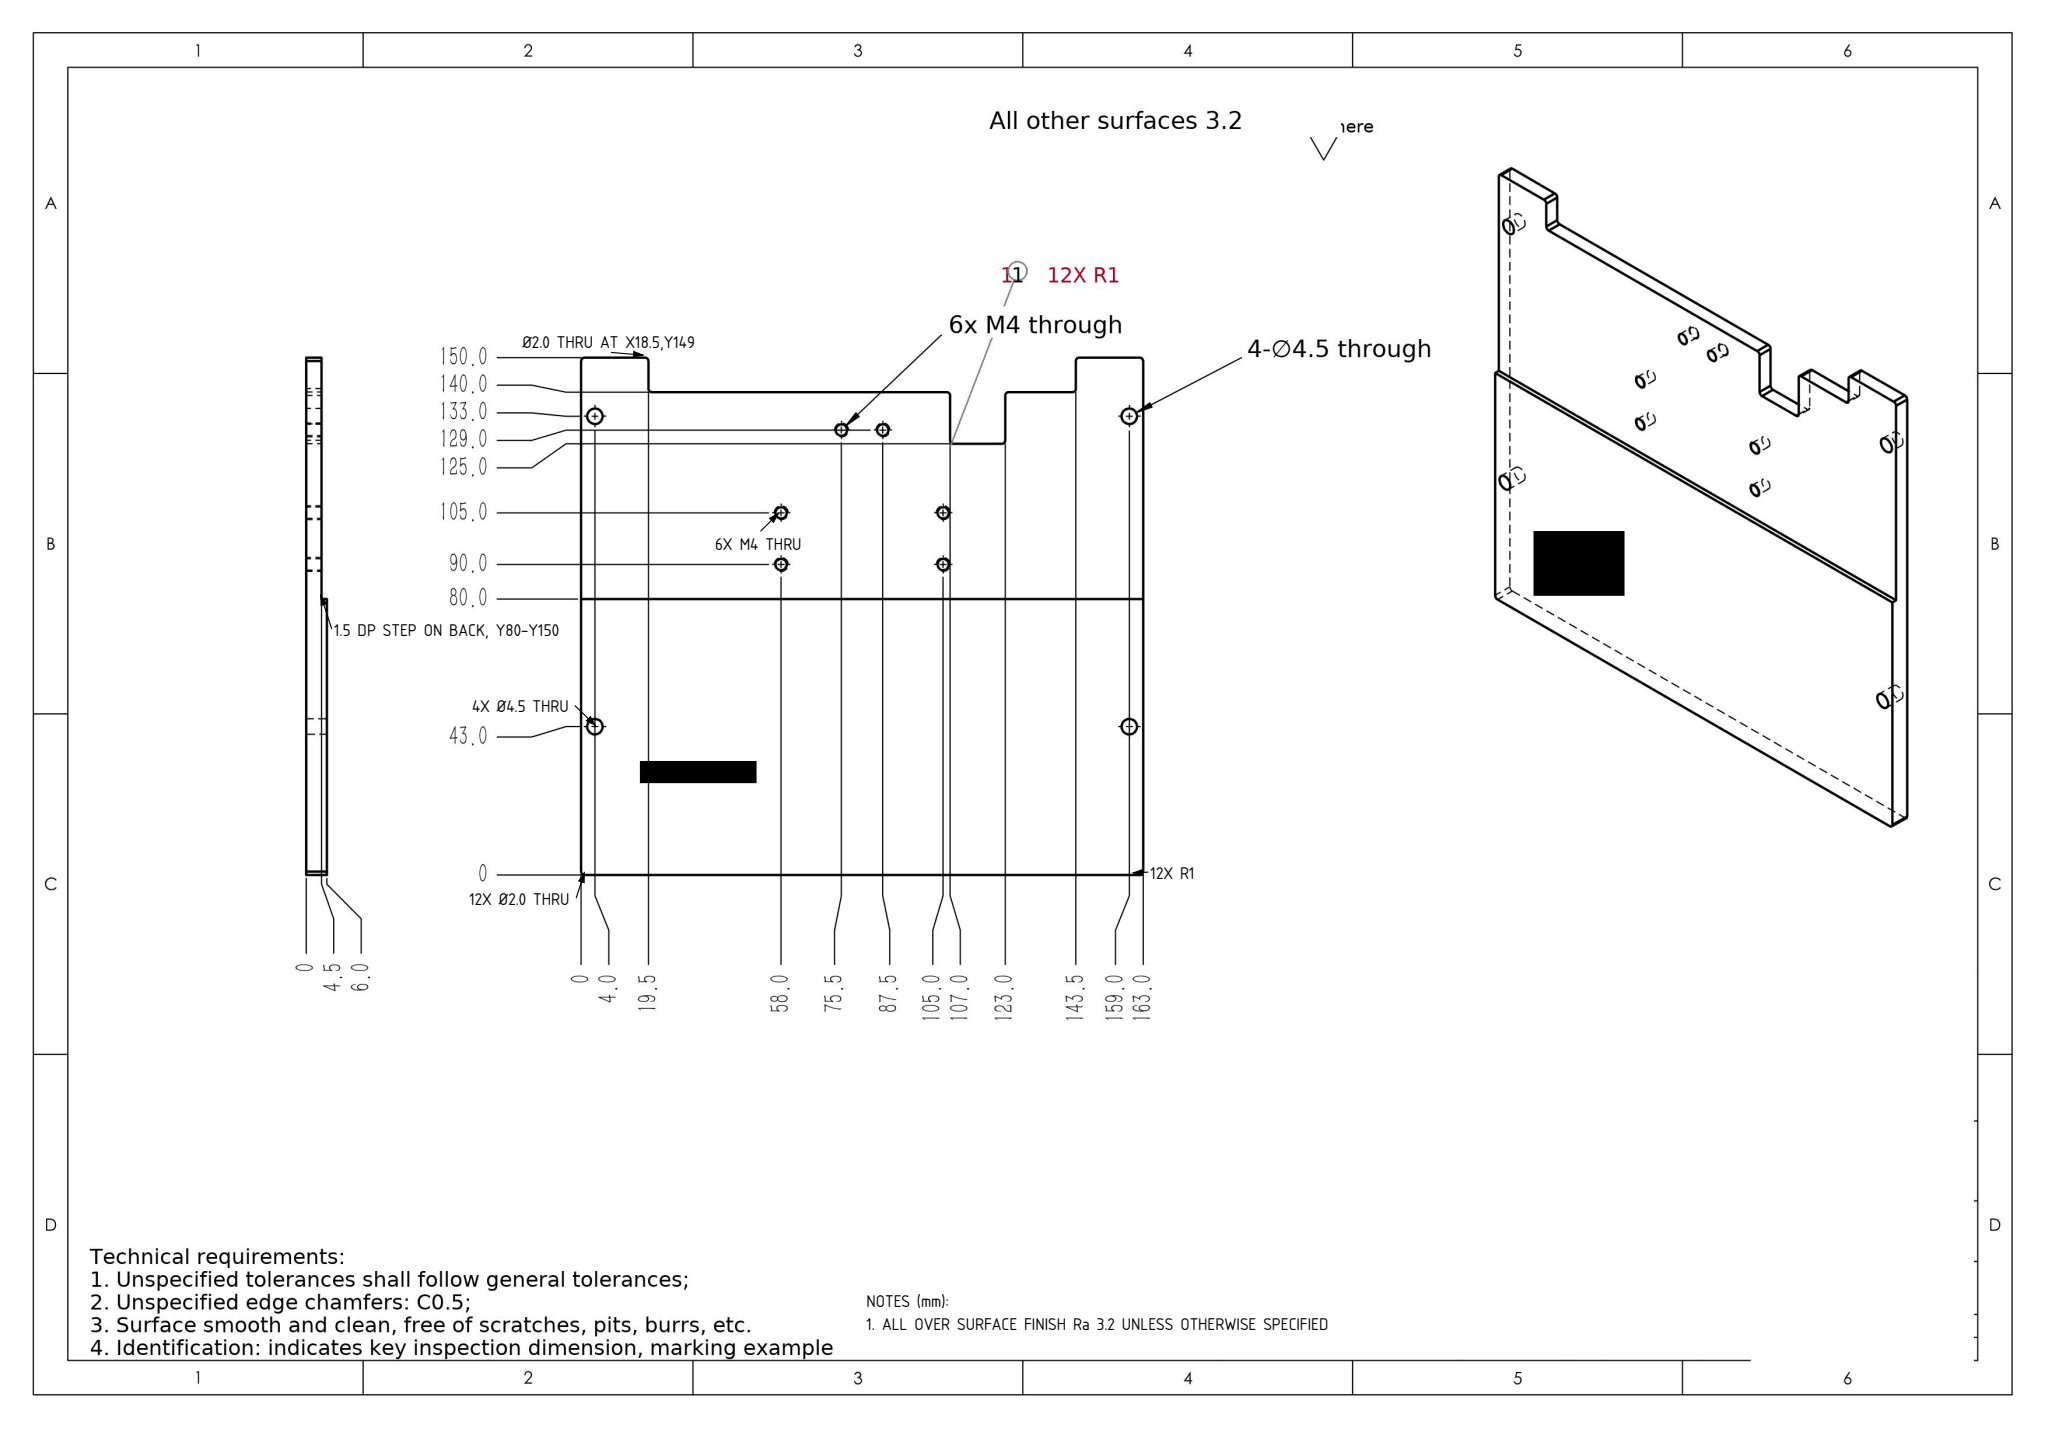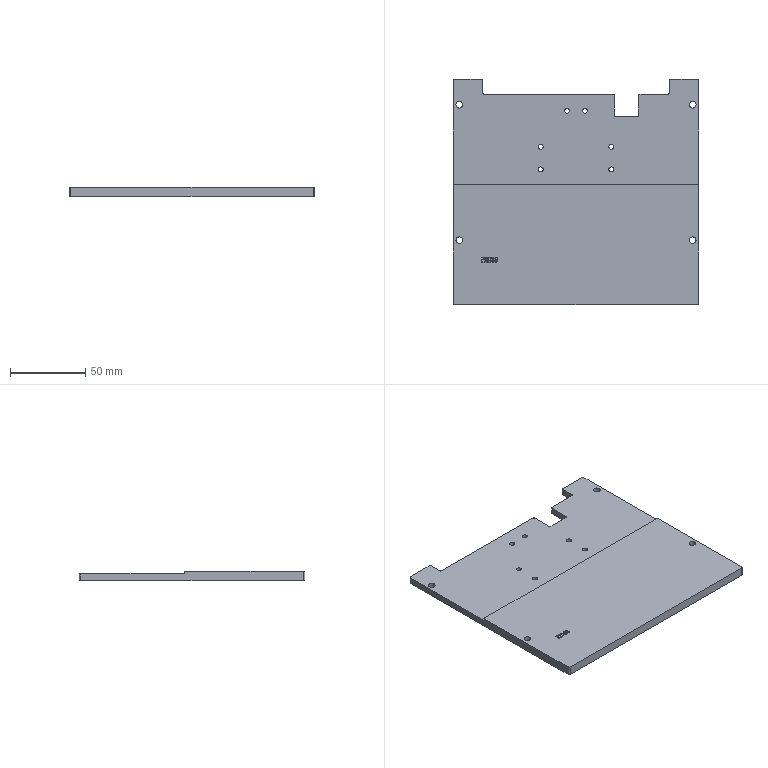Part | SolidWorks | mm | 1 solid | 56 faces | box 163 x 150 x 6 mm | volume 122356 mm3 | cylinder 32 | plane 24 | commonest cylinder face diameters 3.3 x12 2 x12 4.5 x8
Drawing notes:
STEP ON BACK FACE 1.5 DP, FROM Y80.0 TO Y150.0, FULL 163 WIDE (4.5 THK) | from the solid: z planes 0/4.5/6.0; y plane at 80.0 splits 6.0 thk (holes L=6.0 at y=43) from 4.5 thk (holes L=4.5 at y>=90); bbox 163x150x6
12X Ø2.0 THRU - 4 corner holes at (X1.0,Y1.0), (X162.0,Y1.0), (X1.0,Y149.0), (X162.0,Y149.0) from bbox min corner | from the solid: cylinders dia 2.0 axis z at [1,1], [162,1], [1,149], [162,149]
12X Ø2.0 THRU (cont.) - remaining 8 holes at (18.5,149.0), (20.5,141.0), (106.0,139.0), (108.0,126.0), (122.0,126.0), (124.0,139.0), (142.5,141.0), (144.5,149.0) from bbox min corner | from the solid: cylinders dia 2.0 axis z at [18.5,149],[20.5,141],[106,139],[108,126],[122,126],[124,139],[142.5,141],[144.5,149]
ALL OVER SURFACE FINISH Ra 3.2 UNLESS OTHERWISE SPECIFIED | from the solid: no STEP finish data; retains legible sheet value 'All other surfaces 3.2'
12X R1 CORNER FILLETS ON OUTLINE (Ø2.0 FILLET FACES), AT X1.0/Y1.0, X162.0/Y1.0, X1.0/Y149.0, X18.5/Y149.0, X20.5/Y141.0, X106.0/Y139.0, X108.0/Y126.0, X122.0/Y126.0, X124.0/Y139.0, X142.5/Y141.0, X144.5/Y149.0, X162.0/Y149.0 FROM BBOX MIN CORNER | from the solid: cylinders[dia 2.0, axis z] - 12 instances at listed x,y positions
6X M4 THRU (Ø3.3 TAP DRILL, 4.5 DEEP THRU PLATE) AT X58.0/Y90.0, X58.0/Y105.0, X75.5/Y129.0, X87.5/Y129.0, X105.0/Y90.0, X105.0/Y105.0 FROM BBOX MIN CORNER | from the solid: cylinders[3.3, z, length 4.5] at (58,90),(58,105),(75.5,129),(87.5,129),(105,90),(105,105)
4X Ø4.5 THRU AT X4.0/Y43.0, X4.0/Y133.0, X159.0/Y43.0, X159.0/Y133.0 FROM BBOX MIN CORNER | from the solid: cylinders[4.5, z, lengths 6.0 and 4.5] at (4,43),(4,133),(159,43),(159,133)